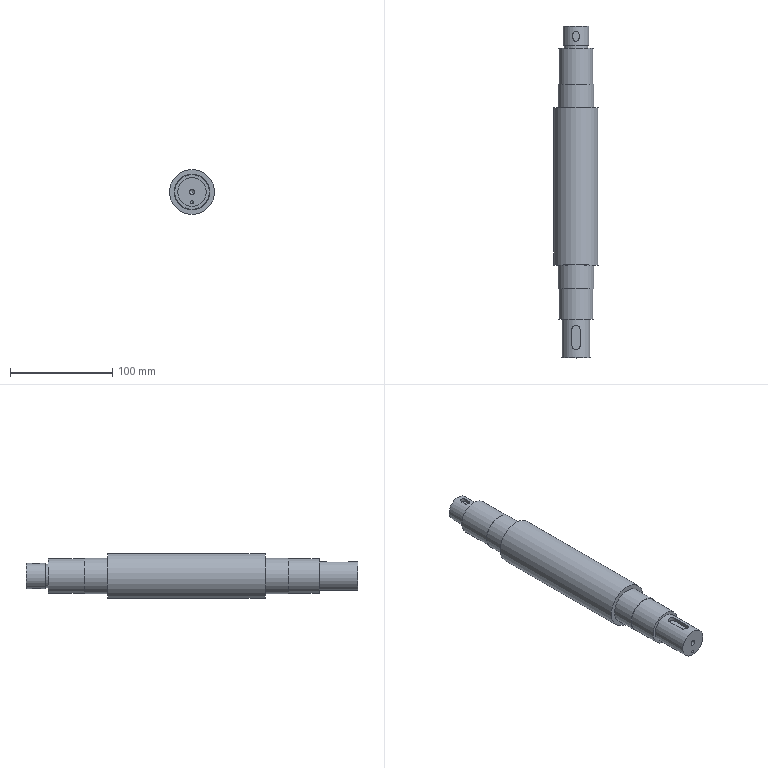Component | NX | SHAFT | 1 solid | 38 faces | volume 369441 mm3 | plane 18 | cylinder 17 | cone 3 | commonest cylinder face diameters 6 x4 34 x2 35 x2 5 x2 8 x2 25 x1 28 x1 23 x1